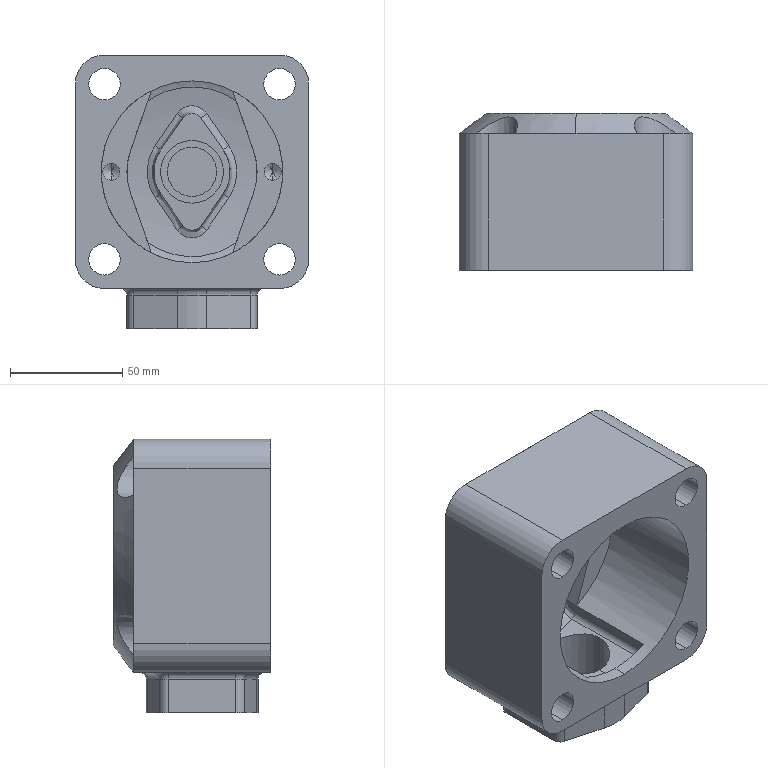Component | SolidWorks | 1-1 | 1 solid | 131 faces | volume 390888 mm3 | cylinder 66 | plane 41 | spline 12 | cone 6 | torus 6 | commonest cylinder face diameters 26 x11 20 x8 14 x8 6 x8 7.5 x4 92 x4 8 x4 10 x3